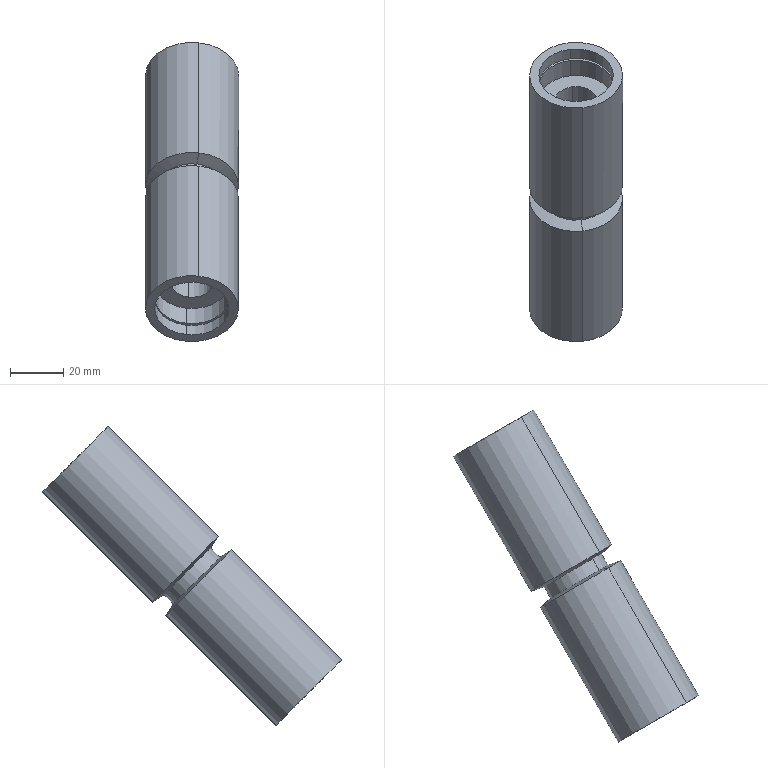Component | SolidWorks | SmallAxisAssembly-1_SmallAxisAssembly1-2_VegetablePressSmallAxisSleeve-1 | 1 solid | 32 faces | box 35.06 x 112.43 x 112.43 mm | volume 79723 mm3 | cylinder 20 | plane 8 | cone 4 | commonest cylinder face diameters 28 x8 30 x4 35 x4 16 x2 25 x2
build123d program:
from build123d import *


with BuildPart() as part:
    # Sketch1 → Revolve1 (revolve)
    with BuildSketch(Plane.XY, mode=Mode.PRIVATE) as revolve1_sk:
        Polygon((-48, 8), (48, 8), (48, 14), (56, 14), (56, 15), (57, 15), (57, 14), (62, 14), (62, 17.5), (3.5, 17.5), (2.5, 12.5), (-2.5, 12.5), (-3.5, 17.5), (-62, 17.5), (-62, 14), (-57, 14), (-57, 15), (-56, 15), (-56, 14), (-48, 14), align=None)
    revolve(revolve1_sk.sketch.rotate(Axis((-52.23, 0, 0), (1, 0, 0)), 90), axis=Axis((-52.23, 0, 0), (1, 0, 0)))


solid = part.part

# Placed as in the assembly
solid = solid.moved(Location((-41.751, 822.318, 226.866), (-134.835, -79.741, -89.832)))
STEP:
#1=CARTESIAN_POINT('',(-1.564,30.402,7.73));
#2=VERTEX_POINT('',#1);
#3=CARTESIAN_POINT('',(-1.726,31.173,6.959));
#4=VERTEX_POINT('',#3);
#5=CARTESIAN_POINT('',(-1.645,30.788,7.345));
#6=DIRECTION('',(-0.0005225,-0.7071,-0.7071));
#7=DIRECTION('',(-0.1474,0.6994,-0.6993));
#8=AXIS2_PLACEMENT_3D('',#5,#6,#7);
#9=CIRCLE('',#8,0.5512);
#10=EDGE_CURVE('',#2,#4,#9,.T.);
#11=ORIENTED_EDGE('',*,*,#10,.F.);
#12=CARTESIAN_POINT('',(-1.564,30.263,7.591));
#13=VERTEX_POINT('',#12);
#14=CARTESIAN_POINT('',(-1.564,30.535,7.863));
#15=DIRECTION('',(-0.0005225,-0.7071,-0.7071));
#16=VECTOR('',#15,39.37);
#17=LINE('',#14,#16);
#18=EDGE_CURVE('',#2,#13,#17,.T.);
#19=ORIENTED_EDGE('',*,*,#18,.T.);
#20=CARTESIAN_POINT('',(-1.726,31.034,6.82));
#21=VERTEX_POINT('',#20);
#22=CARTESIAN_POINT('',(-1.645,30.649,7.206));
#23=DIRECTION('',(-0.0005225,-0.7071,-0.7071));
#24=DIRECTION('',(-0.1474,0.6994,-0.6993));
#25=AXIS2_PLACEMENT_3D('',#22,#23,#24);
#26=CIRCLE('',#25,0.5512);
#27=EDGE_CURVE('',#13,#21,#26,.T.);
#28=ORIENTED_EDGE('',*,*,#27,.T.);
#29=CARTESIAN_POINT('',(-1.726,31.306,7.092));
#30=DIRECTION('',(-0.0005225,-0.7071,-0.7071));
#31=VECTOR('',#30,39.37);
#32=LINE('',#29,#31);
#33=EDGE_CURVE('',#4,#21,#32,.T.);
#34=ORIENTED_EDGE('',*,*,#33,.F.);
#35=EDGE_LOOP('',(#11,#19,#28,#34));
#36=FACE_OUTER_BOUND('',#35,.T.);
#37=CARTESIAN_POINT('',(-1.645,30.921,7.478));
#38=DIRECTION('',(-0.0005225,-0.7071,-0.7071));
#39=DIRECTION('',(-0.1474,0.6994,-0.6993));
#40=AXIS2_PLACEMENT_3D('',#37,#38,#39);
#41=CYLINDRICAL_SURFACE('',#40,0.5512);
#42=ADVANCED_FACE('',(#36),#41,.F.);
#43=CARTESIAN_POINT('',(-1.558,30.403,7.786));
#44=VERTEX_POINT('',#43);
#45=CARTESIAN_POINT('',(-1.732,31.229,6.96));
#46=VERTEX_POINT('',#45);
#47=CARTESIAN_POINT('',(-1.645,30.816,7.373));
#48=DIRECTION('',(-0.0005225,-0.7071,-0.7071));
#49=DIRECTION('',(-0.1474,0.6994,-0.6993));
#50=AXIS2_PLACEMENT_3D('',#47,#48,#49);
#51=CIRCLE('',#50,0.5906);
#52=EDGE_CURVE('',#44,#46,#51,.T.);
#53=ORIENTED_EDGE('',*,*,#52,.F.);
#54=CARTESIAN_POINT('',(-1.558,30.375,7.758));
#55=VERTEX_POINT('',#54);
#56=CARTESIAN_POINT('',(-1.558,30.508,7.891));
#57=DIRECTION('',(-0.0005225,-0.7071,-0.7071));
#58=VECTOR('',#57,39.37);
#59=LINE('',#56,#58);
#60=EDGE_CURVE('',#44,#55,#59,.T.);
#61=ORIENTED_EDGE('',*,*,#60,.T.);
#62=CARTESIAN_POINT('',(-1.732,31.201,6.932));
#63=VERTEX_POINT('',#62);
#64=CARTESIAN_POINT('',(-1.645,30.788,7.345));
#65=DIRECTION('',(-0.0005225,-0.7071,-0.7071));
#66=DIRECTION('',(-0.1474,0.6994,-0.6993));
#67=AXIS2_PLACEMENT_3D('',#64,#65,#66);
#68=CIRCLE('',#67,0.5906);
#69=EDGE_CURVE('',#55,#63,#68,.T.);
#70=ORIENTED_EDGE('',*,*,#69,.T.);
#71=CARTESIAN_POINT('',(-1.732,31.334,7.065));
#72=DIRECTION('',(-0.0005225,-0.7071,-0.7071));
#73=VECTOR('',#72,39.37);
#74=LINE('',#71,#73);
#75=EDGE_CURVE('',#46,#63,#74,.T.);
#76=ORIENTED_EDGE('',*,*,#75,.F.);
#77=EDGE_LOOP('',(#53,#61,#70,#76));
#78=FACE_OUTER_BOUND('',#77,.T.);
#79=CARTESIAN_POINT('',(-1.645,30.921,7.478));
#80=DIRECTION('',(-0.0005225,-0.7071,-0.7071));
#81=DIRECTION('',(-0.1474,0.6994,-0.6993));
#82=AXIS2_PLACEMENT_3D('',#79,#80,#81);
#83=CYLINDRICAL_SURFACE('',#82,0.5906);
#84=ADVANCED_FACE('',(#78),#83,.F.);
#85=CARTESIAN_POINT('',(-1.563,30.653,7.981));
#86=VERTEX_POINT('',#85);
#87=CARTESIAN_POINT('',(-1.726,31.424,7.21));
#88=VERTEX_POINT('',#87);
#89=CARTESIAN_POINT('',(-1.645,31.038,7.595));
#90=DIRECTION('',(-0.0005225,-0.7071,-0.7071));
#91=DIRECTION('',(-0.1474,0.6994,-0.6993));
#92=AXIS2_PLACEMENT_3D('',#89,#90,#91);
#93=CIRCLE('',#92,0.5512);
#94=EDGE_CURVE('',#86,#88,#93,.T.);
#95=ORIENTED_EDGE('',*,*,#94,.F.);
#96=CARTESIAN_POINT('',(-1.564,30.43,7.758));
#97=VERTEX_POINT('',#96);
#98=CARTESIAN_POINT('',(-1.564,30.535,7.863));
#99=DIRECTION('',(-0.0005225,-0.7071,-0.7071));
#100=VECTOR('',#99,39.37);
#101=LINE('',#98,#100);
#102=EDGE_CURVE('',#86,#97,#101,.T.);
#103=ORIENTED_EDGE('',*,*,#102,.T.);
#104=CARTESIAN_POINT('',(-1.726,31.201,6.987));
#105=VERTEX_POINT('',#104);
#106=CARTESIAN_POINT('',(-1.645,30.816,7.373));
#107=DIRECTION('',(-0.0005225,-0.7071,-0.7071));
#108=DIRECTION('',(-0.1474,0.6994,-0.6993));
#109=AXIS2_PLACEMENT_3D('',#106,#107,#108);
#110=CIRCLE('',#109,0.5512);
#111=EDGE_CURVE('',#97,#105,#110,.T.);
#112=ORIENTED_EDGE('',*,*,#111,.T.);
#113=CARTESIAN_POINT('',(-1.726,31.306,7.092));
#114=DIRECTION('',(-0.0005225,-0.7071,-0.7071));
#115=VECTOR('',#114,39.37);
#116=LINE('',#113,#115);
#117=EDGE_CURVE('',#88,#105,#116,.T.);
#118=ORIENTED_EDGE('',*,*,#117,.F.);
#119=EDGE_LOOP('',(#95,#103,#112,#118));
#120=FACE_OUTER_BOUND('',#119,.T.);
#121=CARTESIAN_POINT('',(-1.645,30.921,7.478));
#122=DIRECTION('',(-0.0005225,-0.7071,-0.7071));
#123=DIRECTION('',(-0.1474,0.6994,-0.6993));
#124=AXIS2_PLACEMENT_3D('',#121,#122,#123);
#125=CYLINDRICAL_SURFACE('',#124,0.5512);
#126=ADVANCED_FACE('',(#120),#125,.F.);
#127=CARTESIAN_POINT('',(-1.596,33.491,10.488));
#128=VERTEX_POINT('',#127);
#129=CARTESIAN_POINT('',(-1.689,33.931,10.048));
#130=VERTEX_POINT('',#129);
#131=CARTESIAN_POINT('',(-1.643,33.711,10.268));
#132=DIRECTION('',(-0.0005225,-0.7071,-0.7071));
#133=DIRECTION('',(-0.1474,0.6994,-0.6993));
#134=AXIS2_PLACEMENT_3D('',#131,#132,#133);
#135=CIRCLE('',#134,0.315);
#136=EDGE_CURVE('',#128,#130,#135,.T.);
#137=ORIENTED_EDGE('',*,*,#136,.F.);
#138=CARTESIAN_POINT('',(-1.598,30.818,7.816));
#139=VERTEX_POINT('',#138);
#140=CARTESIAN_POINT('',(-1.598,30.7,7.698));
#141=DIRECTION('',(-0.0005225,-0.7071,-0.7071));
#142=VECTOR('',#141,39.37);
#143=LINE('',#140,#142);
#144=EDGE_CURVE('',#128,#139,#143,.T.);
#145=ORIENTED_EDGE('',*,*,#144,.T.);
#146=CARTESIAN_POINT('',(-1.691,31.259,7.375));
#147=VERTEX_POINT('',#146);
#148=CARTESIAN_POINT('',(-1.645,31.038,7.595));
#149=DIRECTION('',(-0.0005225,-0.7071,-0.7071));
#150=DIRECTION('',(-0.1474,0.6994,-0.6993));
#151=AXIS2_PLACEMENT_3D('',#148,#149,#150);
#152=CIRCLE('',#151,0.315);
#153=EDGE_CURVE('',#139,#147,#152,.T.);
#154=ORIENTED_EDGE('',*,*,#153,.T.);
#155=CARTESIAN_POINT('',(-1.691,31.141,7.257));
#156=DIRECTION('',(-0.0005225,-0.7071,-0.7071));
#157=VECTOR('',#156,39.37);
#158=LINE('',#155,#157);
#159=EDGE_CURVE('',#130,#147,#158,.T.);
#160=ORIENTED_EDGE('',*,*,#159,.F.);
#161=EDGE_LOOP('',(#137,#145,#154,#160));
#162=FACE_OUTER_BOUND('',#161,.T.);
#163=CARTESIAN_POINT('',(-1.645,30.921,7.478));
#164=DIRECTION('',(-0.0005225,-0.7071,-0.7071));
#165=DIRECTION('',(-0.1474,0.6994,-0.6993));
#166=AXIS2_PLACEMENT_3D('',#163,#164,#165);
#167=CYLINDRICAL_SURFACE('',#166,0.315);
#168=ADVANCED_FACE('',(#162),#167,.F.);
#169=CARTESIAN_POINT('',(-1.561,33.548,10.876));
#170=VERTEX_POINT('',#169);
#171=CARTESIAN_POINT('',(-1.724,34.319,10.105));
#172=VERTEX_POINT('',#171);
#173=CARTESIAN_POINT('',(-1.643,33.934,10.491));
#174=DIRECTION('',(-0.0005225,-0.7071,-0.7071));
#175=DIRECTION('',(-0.1474,0.6994,-0.6993));
#176=AXIS2_PLACEMENT_3D('',#173,#174,#175);
#177=CIRCLE('',#176,0.5512);
#178=EDGE_CURVE('',#170,#172,#177,.T.);
#179=ORIENTED_EDGE('',*,*,#178,.F.);
#180=CARTESIAN_POINT('',(-1.562,33.325,10.653));
#181=VERTEX_POINT('',#180);
#182=CARTESIAN_POINT('',(-1.564,30.535,7.863));
#183=DIRECTION('',(-0.0005225,-0.7071,-0.7071));
#184=VECTOR('',#183,39.37);
#185=LINE('',#182,#184);
#186=EDGE_CURVE('',#170,#181,#185,.T.);
#187=ORIENTED_EDGE('',*,*,#186,.T.);
#188=CARTESIAN_POINT('',(-1.724,34.097,9.883));
#189=VERTEX_POINT('',#188);
#190=CARTESIAN_POINT('',(-1.643,33.711,10.268));
#191=DIRECTION('',(-0.0005225,-0.7071,-0.7071));
#192=DIRECTION('',(-0.1474,0.6994,-0.6993));
#193=AXIS2_PLACEMENT_3D('',#190,#191,#192);
#194=CIRCLE('',#193,0.5512);
#195=EDGE_CURVE('',#181,#189,#194,.T.);
#196=ORIENTED_EDGE('',*,*,#195,.T.);
#197=CARTESIAN_POINT('',(-1.726,31.306,7.092));
#198=DIRECTION('',(-0.0005225,-0.7071,-0.7071));
#199=VECTOR('',#198,39.37);
#200=LINE('',#197,#199);
#201=EDGE_CURVE('',#172,#189,#200,.T.);
#202=ORIENTED_EDGE('',*,*,#201,.F.);
#203=EDGE_LOOP('',(#179,#187,#196,#202));
#204=FACE_OUTER_BOUND('',#203,.T.);
#205=CARTESIAN_POINT('',(-1.645,30.921,7.478));
#206=DIRECTION('',(-0.0005225,-0.7071,-0.7071));
#207=DIRECTION('',(-0.1474,0.6994,-0.6993));
#208=AXIS2_PLACEMENT_3D('',#205,#206,#207);
#209=CYLINDRICAL_SURFACE('',#208,0.5512);
#210=ADVANCED_FACE('',(#204),#209,.F.);
#211=CARTESIAN_POINT('',(-1.556,33.548,10.932));
#212=VERTEX_POINT('',#211);
#213=CARTESIAN_POINT('',(-1.73,34.375,10.106));
#214=VERTEX_POINT('',#213);
#215=CARTESIAN_POINT('',(-1.643,33.962,10.519));
#216=DIRECTION('',(-0.0005225,-0.7071,-0.7071));
#217=DIRECTION('',(-0.1474,0.6994,-0.6993));
#218=AXIS2_PLACEMENT_3D('',#215,#216,#217);
#219=CIRCLE('',#218,0.5906);
#220=EDGE_CURVE('',#212,#214,#219,.T.);
#221=ORIENTED_EDGE('',*,*,#220,.F.);
#222=CARTESIAN_POINT('',(-1.556,33.521,10.904));
#223=VERTEX_POINT('',#222);
#224=CARTESIAN_POINT('',(-1.558,30.508,7.891));
#225=DIRECTION('',(-0.0005225,-0.7071,-0.7071));
#226=VECTOR('',#225,39.37);
#227=LINE('',#224,#226);
#228=EDGE_CURVE('',#212,#223,#227,.T.);
#229=ORIENTED_EDGE('',*,*,#228,.T.);
#230=CARTESIAN_POINT('',(-1.73,34.347,10.078));
#231=VERTEX_POINT('',#230);
#232=CARTESIAN_POINT('',(-1.643,33.934,10.491));
#233=DIRECTION('',(-0.0005225,-0.7071,-0.7071));
#234=DIRECTION('',(-0.1474,0.6994,-0.6993));
#235=AXIS2_PLACEMENT_3D('',#232,#233,#234);
#236=CIRCLE('',#235,0.5906);
#237=EDGE_CURVE('',#223,#231,#236,.T.);
#238=ORIENTED_EDGE('',*,*,#237,.T.);
#239=CARTESIAN_POINT('',(-1.732,31.334,7.065));
#240=DIRECTION('',(-0.0005225,-0.7071,-0.7071));
#241=VECTOR('',#240,39.37);
#242=LINE('',#239,#241);
#243=EDGE_CURVE('',#214,#231,#242,.T.);
#244=ORIENTED_EDGE('',*,*,#243,.F.);
#245=EDGE_LOOP('',(#221,#229,#238,#244));
#246=FACE_OUTER_BOUND('',#245,.T.);
#247=CARTESIAN_POINT('',(-1.645,30.921,7.478));
#248=DIRECTION('',(-0.0005225,-0.7071,-0.7071));
#249=DIRECTION('',(-0.1474,0.6994,-0.6993));
#250=AXIS2_PLACEMENT_3D('',#247,#248,#249);
#251=CYLINDRICAL_SURFACE('',#250,0.5906);
#252=ADVANCED_FACE('',(#246),#251,.F.);
#253=CARTESIAN_POINT('',(-1.561,33.715,11.043));
#254=VERTEX_POINT('',#253);
#255=CARTESIAN_POINT('',(-1.724,34.486,10.272));
#256=VERTEX_POINT('',#255);
#257=CARTESIAN_POINT('',(-1.642,34.101,10.658));
#258=DIRECTION('',(-0.0005225,-0.7071,-0.7071));
#259=DIRECTION('',(-0.1474,0.6994,-0.6993));
#260=AXIS2_PLACEMENT_3D('',#257,#258,#259);
#261=CIRCLE('',#260,0.5512);
#262=EDGE_CURVE('',#254,#256,#261,.T.);
#263=ORIENTED_EDGE('',*,*,#262,.F.);
#264=CARTESIAN_POINT('',(-1.561,33.576,10.904));
#265=VERTEX_POINT('',#264);
#266=CARTESIAN_POINT('',(-1.564,30.535,7.863));
#267=DIRECTION('',(-0.0005225,-0.7071,-0.7071));
#268=VECTOR('',#267,39.37);
#269=LINE('',#266,#268);
#270=EDGE_CURVE('',#254,#265,#269,.T.);
#271=ORIENTED_EDGE('',*,*,#270,.T.);
#272=CARTESIAN_POINT('',(-1.724,34.347,10.133));
#273=VERTEX_POINT('',#272);
#274=CARTESIAN_POINT('',(-1.643,33.962,10.519));
#275=DIRECTION('',(-0.0005225,-0.7071,-0.7071));
#276=DIRECTION('',(-0.1474,0.6994,-0.6993));
#277=AXIS2_PLACEMENT_3D('',#274,#275,#276);
#278=CIRCLE('',#277,0.5512);
#279=EDGE_CURVE('',#265,#273,#278,.T.);
#280=ORIENTED_EDGE('',*,*,#279,.T.);
#281=CARTESIAN_POINT('',(-1.726,31.306,7.092));
#282=DIRECTION('',(-0.0005225,-0.7071,-0.7071));
#283=VECTOR('',#282,39.37);
#284=LINE('',#281,#283);
#285=EDGE_CURVE('',#256,#273,#284,.T.);
#286=ORIENTED_EDGE('',*,*,#285,.F.);
#287=EDGE_LOOP('',(#263,#271,#280,#286));
#288=FACE_OUTER_BOUND('',#287,.T.);
#289=CARTESIAN_POINT('',(-1.645,30.921,7.478));
#290=DIRECTION('',(-0.0005225,-0.7071,-0.7071));
#291=DIRECTION('',(-0.1474,0.6994,-0.6993));
#292=AXIS2_PLACEMENT_3D('',#289,#290,#291);
#293=CYLINDRICAL_SURFACE('',#292,0.5512);
#294=ADVANCED_FACE('',(#288),#293,.F.);
#295=CARTESIAN_POINT('',(-1.744,34.583,10.176));
#296=VERTEX_POINT('',#295);
#297=CARTESIAN_POINT('',(-1.541,33.619,11.14));
#298=VERTEX_POINT('',#297);
#299=CARTESIAN_POINT('',(-1.642,34.101,10.658));
#300=DIRECTION('',(-0.0005225,-0.7071,-0.7071));
#301=DIRECTION('',(-0.1474,0.6994,-0.6993));
#302=AXIS2_PLACEMENT_3D('',#299,#300,#301);
#303=CIRCLE('',#302,0.689);
#304=EDGE_CURVE('',#296,#298,#303,.T.);
#305=ORIENTED_EDGE('',*,*,#304,.T.);
#306=CARTESIAN_POINT('',(-1.542,31.99,9.511));
#307=VERTEX_POINT('',#306);
#308=CARTESIAN_POINT('',(-1.543,30.439,7.96));
#309=DIRECTION('',(-0.0005225,-0.7071,-0.7071));
#310=VECTOR('',#309,39.37);
#311=LINE('',#308,#310);
#312=EDGE_CURVE('',#298,#307,#311,.T.);
#313=ORIENTED_EDGE('',*,*,#312,.T.);
#314=CARTESIAN_POINT('',(-1.745,32.954,8.547));
#315=VERTEX_POINT('',#314);
#316=CARTESIAN_POINT('',(-1.644,32.472,9.029));
#317=DIRECTION('',(-0.0005225,-0.7071,-0.7071));
#318=DIRECTION('',(-0.1474,0.6994,-0.6993));
#319=AXIS2_PLACEMENT_3D('',#316,#317,#318);
#320=CIRCLE('',#319,0.689);
#321=EDGE_CURVE('',#315,#307,#320,.T.);
#322=ORIENTED_EDGE('',*,*,#321,.F.);
#323=CARTESIAN_POINT('',(-1.746,31.403,6.996));
#324=DIRECTION('',(-0.0005225,-0.7071,-0.7071));
#325=VECTOR('',#324,39.37);
#326=LINE('',#323,#325);
#327=EDGE_CURVE('',#296,#315,#326,.T.);
#328=ORIENTED_EDGE('',*,*,#327,.F.);
#329=EDGE_LOOP('',(#305,#313,#322,#328));
#330=FACE_OUTER_BOUND('',#329,.T.);
#331=CARTESIAN_POINT('',(-1.645,30.921,7.478));
#332=DIRECTION('',(-0.0005225,-0.7071,-0.7071));
#333=DIRECTION('',(-0.1474,0.6994,-0.6993));
#334=AXIS2_PLACEMENT_3D('',#331,#332,#333);
#335=CYLINDRICAL_SURFACE('',#334,0.689);
#336=ADVANCED_FACE('',(#330),#335,.T.);
#337=CARTESIAN_POINT('',(-1.716,32.789,8.657));
#338=VERTEX_POINT('',#337);
#339=CARTESIAN_POINT('',(-1.571,32.1,9.345));
#340=VERTEX_POINT('',#339);
#341=CARTESIAN_POINT('',(-1.644,32.444,9.001));
#342=DIRECTION('',(-0.0005225,-0.7071,-0.7071));
#343=DIRECTION('',(-0.1474,0.6994,-0.6993));
#344=AXIS2_PLACEMENT_3D('',#341,#342,#343);
#345=CIRCLE('',#344,0.4921);
#346=EDGE_CURVE('',#338,#340,#345,.T.);
#347=ORIENTED_EDGE('',*,*,#346,.F.);
#348=CARTESIAN_POINT('',(-1.745,32.954,8.547));
#349=DIRECTION('',(-0.1444,0.8245,-0.5471));
#350=VECTOR('',#349,39.37);
#351=LINE('',#348,#350);
#352=EDGE_CURVE('',#338,#315,#351,.T.);
#353=ORIENTED_EDGE('',*,*,#352,.T.);
#354=ORIENTED_EDGE('',*,*,#321,.T.);
#355=CARTESIAN_POINT('',(-1.542,31.99,9.511));
#356=DIRECTION('',(0.1447,-0.5472,0.8244));
#357=VECTOR('',#356,39.37);
#358=LINE('',#355,#357);
#359=EDGE_CURVE('',#340,#307,#358,.T.);
#360=ORIENTED_EDGE('',*,*,#359,.F.);
#361=EDGE_LOOP('',(#347,#353,#354,#360));
#362=FACE_OUTER_BOUND('',#361,.T.);
#363=CARTESIAN_POINT('',(-1.644,32.472,9.029));
#364=DIRECTION('',(0.0005225,0.7071,0.7071));
#365=DIRECTION('',(0.1474,-0.6994,0.6993));
#366=AXIS2_PLACEMENT_3D('',#363,#364,#365);
#367=CONICAL_SURFACE('',#366,0.689,1.373);
#368=ADVANCED_FACE('',(#362),#367,.T.);
#369=ORIENTED_EDGE('',*,*,#346,.T.);
#370=CARTESIAN_POINT('',(-1.571,31.961,9.206));
#371=VERTEX_POINT('',#370);
#372=CARTESIAN_POINT('',(-1.572,30.576,7.822));
#373=DIRECTION('',(-0.0005225,-0.7071,-0.7071));
#374=VECTOR('',#373,39.37);
#375=LINE('',#372,#374);
#376=EDGE_CURVE('',#340,#371,#375,.T.);
#377=ORIENTED_EDGE('',*,*,#376,.T.);
#378=CARTESIAN_POINT('',(-1.716,32.649,8.518));
#379=VERTEX_POINT('',#378);
#380=CARTESIAN_POINT('',(-1.644,32.305,8.862));
#381=DIRECTION('',(-0.0005225,-0.7071,-0.7071));
#382=DIRECTION('',(-0.1474,0.6994,-0.6993));
#383=AXIS2_PLACEMENT_3D('',#380,#381,#382);
#384=CIRCLE('',#383,0.4921);
#385=EDGE_CURVE('',#379,#371,#384,.T.);
#386=ORIENTED_EDGE('',*,*,#385,.F.);
#387=CARTESIAN_POINT('',(-1.717,31.265,7.134));
#388=DIRECTION('',(-0.0005225,-0.7071,-0.7071));
#389=VECTOR('',#388,39.37);
#390=LINE('',#387,#389);
#391=EDGE_CURVE('',#338,#379,#390,.T.);
#392=ORIENTED_EDGE('',*,*,#391,.F.);
#393=EDGE_LOOP('',(#369,#377,#386,#392));
#394=FACE_OUTER_BOUND('',#393,.T.);
#395=CARTESIAN_POINT('',(-1.645,30.921,7.478));
#396=DIRECTION('',(-0.0005225,-0.7071,-0.7071));
#397=DIRECTION('',(-0.1474,0.6994,-0.6993));
#398=AXIS2_PLACEMENT_3D('',#395,#396,#397);
#399=CYLINDRICAL_SURFACE('',#398,0.4921);
#400=ADVANCED_FACE('',(#394),#399,.T.);
#401=ORIENTED_EDGE('',*,*,#385,.T.);
#402=CARTESIAN_POINT('',(-1.542,31.795,9.316));
#403=VERTEX_POINT('',#402);
#404=CARTESIAN_POINT('',(-1.571,31.961,9.206));
#405=DIRECTION('',(0.1444,-0.8245,0.5471));
#406=VECTOR('',#405,39.37);
#407=LINE('',#404,#406);
#408=EDGE_CURVE('',#371,#403,#407,.T.);
#409=ORIENTED_EDGE('',*,*,#408,.T.);
#410=CARTESIAN_POINT('',(-1.745,32.759,8.352));
#411=VERTEX_POINT('',#410);
#412=CARTESIAN_POINT('',(-1.644,32.277,8.834));
#413=DIRECTION('',(-0.0005225,-0.7071,-0.7071));
#414=DIRECTION('',(-0.1474,0.6994,-0.6993));
#415=AXIS2_PLACEMENT_3D('',#412,#413,#414);
#416=CIRCLE('',#415,0.689);
#417=EDGE_CURVE('',#411,#403,#416,.T.);
#418=ORIENTED_EDGE('',*,*,#417,.F.);
#419=CARTESIAN_POINT('',(-1.716,32.649,8.518));
#420=DIRECTION('',(-0.1447,0.5472,-0.8244));
#421=VECTOR('',#420,39.37);
#422=LINE('',#419,#421);
#423=EDGE_CURVE('',#379,#411,#422,.T.);
#424=ORIENTED_EDGE('',*,*,#423,.F.);
#425=EDGE_LOOP('',(#401,#409,#418,#424));
#426=FACE_OUTER_BOUND('',#425,.T.);
#427=CARTESIAN_POINT('',(-1.644,32.305,8.862));
#428=DIRECTION('',(-0.0005225,-0.7071,-0.7071));
#429=DIRECTION('',(-0.1474,0.6994,-0.6993));
#430=AXIS2_PLACEMENT_3D('',#427,#428,#429);
#431=CONICAL_SURFACE('',#430,0.4921,1.373);
#432=ADVANCED_FACE('',(#426),#431,.T.);
#433=ORIENTED_EDGE('',*,*,#417,.T.);
#434=CARTESIAN_POINT('',(-1.543,30.167,7.688));
#435=VERTEX_POINT('',#434);
#436=CARTESIAN_POINT('',(-1.543,30.439,7.96));
#437=DIRECTION('',(-0.0005225,-0.7071,-0.7071));
#438=VECTOR('',#437,39.37);
#439=LINE('',#436,#438);
#440=EDGE_CURVE('',#403,#435,#439,.T.);
#441=ORIENTED_EDGE('',*,*,#440,.T.);
#442=CARTESIAN_POINT('',(-1.747,31.131,6.724));
#443=VERTEX_POINT('',#442);
#444=CARTESIAN_POINT('',(-1.645,30.649,7.206));
#445=DIRECTION('',(-0.0005225,-0.7071,-0.7071));
#446=DIRECTION('',(-0.1474,0.6994,-0.6993));
#447=AXIS2_PLACEMENT_3D('',#444,#445,#446);
#448=CIRCLE('',#447,0.689);
#449=EDGE_CURVE('',#443,#435,#448,.T.);
#450=ORIENTED_EDGE('',*,*,#449,.F.);
#451=CARTESIAN_POINT('',(-1.746,31.403,6.996));
#452=DIRECTION('',(-0.0005225,-0.7071,-0.7071));
#453=VECTOR('',#452,39.37);
#454=LINE('',#451,#453);
#455=EDGE_CURVE('',#411,#443,#454,.T.);
#456=ORIENTED_EDGE('',*,*,#455,.F.);
#457=EDGE_LOOP('',(#433,#441,#450,#456));
#458=FACE_OUTER_BOUND('',#457,.T.);
#459=CARTESIAN_POINT('',(-1.645,30.921,7.478));
#460=DIRECTION('',(-0.0005225,-0.7071,-0.7071));
#461=DIRECTION('',(-0.1474,0.6994,-0.6993));
#462=AXIS2_PLACEMENT_3D('',#459,#460,#461);
#463=CYLINDRICAL_SURFACE('',#462,0.689);
#464=ADVANCED_FACE('',(#458),#463,.T.);
#465=ORIENTED_EDGE('',*,*,#440,.F.);
#466=CARTESIAN_POINT('',(-1.644,32.277,8.834));
#467=DIRECTION('',(-0.0005225,-0.7071,-0.7071));
#468=DIRECTION('',(-0.1474,0.6994,-0.6993));
#469=AXIS2_PLACEMENT_3D('',#466,#467,#468);
#470=CIRCLE('',#469,0.689);
#471=EDGE_CURVE('',#403,#411,#470,.T.);
#472=ORIENTED_EDGE('',*,*,#471,.T.);
#473=ORIENTED_EDGE('',*,*,#455,.T.);
#474=CARTESIAN_POINT('',(-1.645,30.649,7.206));
#475=DIRECTION('',(-0.0005225,-0.7071,-0.7071));
#476=DIRECTION('',(-0.1474,0.6994,-0.6993));
#477=AXIS2_PLACEMENT_3D('',#474,#475,#476);
#478=CIRCLE('',#477,0.689);
#479=EDGE_CURVE('',#435,#443,#478,.T.);
#480=ORIENTED_EDGE('',*,*,#479,.F.);
#481=EDGE_LOOP('',(#465,#472,#473,#480));
#482=FACE_OUTER_BOUND('',#481,.T.);
#483=CARTESIAN_POINT('',(-1.645,30.921,7.478));
#484=DIRECTION('',(-0.0005225,-0.7071,-0.7071));
#485=DIRECTION('',(-0.1474,0.6994,-0.6993));
#486=AXIS2_PLACEMENT_3D('',#483,#484,#485);
#487=CYLINDRICAL_SURFACE('',#486,0.689);
#488=ADVANCED_FACE('',(#482),#487,.T.);
#489=ORIENTED_EDGE('',*,*,#408,.F.);
#490=CARTESIAN_POINT('',(-1.644,32.305,8.862));
#491=DIRECTION('',(-0.0005225,-0.7071,-0.7071));
#492=DIRECTION('',(-0.1474,0.6994,-0.6993));
#493=AXIS2_PLACEMENT_3D('',#490,#491,#492);
#494=CIRCLE('',#493,0.4921);
#495=EDGE_CURVE('',#371,#379,#494,.T.);
#496=ORIENTED_EDGE('',*,*,#495,.T.);
#497=ORIENTED_EDGE('',*,*,#423,.T.);
#498=ORIENTED_EDGE('',*,*,#471,.F.);
#499=EDGE_LOOP('',(#489,#496,#497,#498));
#500=FACE_OUTER_BOUND('',#499,.T.);
#501=CARTESIAN_POINT('',(-1.644,32.305,8.862));
#502=DIRECTION('',(-0.0005225,-0.7071,-0.7071));
#503=DIRECTION('',(-0.1474,0.6994,-0.6993));
#504=AXIS2_PLACEMENT_3D('',#501,#502,#503);
#505=CONICAL_SURFACE('',#504,0.4921,1.373);
#506=ADVANCED_FACE('',(#500),#505,.T.);
#507=ORIENTED_EDGE('',*,*,#376,.F.);
#508=CARTESIAN_POINT('',(-1.644,32.444,9.001));
#509=DIRECTION('',(-0.0005225,-0.7071,-0.7071));
#510=DIRECTION('',(-0.1474,0.6994,-0.6993));
#511=AXIS2_PLACEMENT_3D('',#508,#509,#510);
#512=CIRCLE('',#511,0.4921);
#513=EDGE_CURVE('',#340,#338,#512,.T.);
#514=ORIENTED_EDGE('',*,*,#513,.T.);
#515=ORIENTED_EDGE('',*,*,#391,.T.);
#516=ORIENTED_EDGE('',*,*,#495,.F.);
#517=EDGE_LOOP('',(#507,#514,#515,#516));
#518=FACE_OUTER_BOUND('',#517,.T.);
#519=CARTESIAN_POINT('',(-1.645,30.921,7.478));
#520=DIRECTION('',(-0.0005225,-0.7071,-0.7071));
#521=DIRECTION('',(-0.1474,0.6994,-0.6993));
#522=AXIS2_PLACEMENT_3D('',#519,#520,#521);
#523=CYLINDRICAL_SURFACE('',#522,0.4921);
#524=ADVANCED_FACE('',(#518),#523,.T.);
#525=ORIENTED_EDGE('',*,*,#352,.F.);
#526=ORIENTED_EDGE('',*,*,#513,.F.);
#527=ORIENTED_EDGE('',*,*,#359,.T.);
#528=CARTESIAN_POINT('',(-1.644,32.472,9.029));
#529=DIRECTION('',(-0.0005225,-0.7071,-0.7071));
#530=DIRECTION('',(-0.1474,0.6994,-0.6993));
#531=AXIS2_PLACEMENT_3D('',#528,#529,#530);
#532=CIRCLE('',#531,0.689);
#533=EDGE_CURVE('',#307,#315,#532,.T.);
#534=ORIENTED_EDGE('',*,*,#533,.T.);
#535=EDGE_LOOP('',(#525,#526,#527,#534));
#536=FACE_OUTER_BOUND('',#535,.T.);
#537=CARTESIAN_POINT('',(-1.644,32.472,9.029));
#538=DIRECTION('',(0.0005225,0.7071,0.7071));
#539=DIRECTION('',(0.1474,-0.6994,0.6993));
#540=AXIS2_PLACEMENT_3D('',#537,#538,#539);
#541=CONICAL_SURFACE('',#540,0.689,1.373);
#542=ADVANCED_FACE('',(#536),#541,.T.);
#543=ORIENTED_EDGE('',*,*,#312,.F.);
#544=CARTESIAN_POINT('',(-1.642,34.101,10.658));
#545=DIRECTION('',(-0.0005225,-0.7071,-0.7071));
#546=DIRECTION('',(-0.1474,0.6994,-0.6993));
#547=AXIS2_PLACEMENT_3D('',#544,#545,#546);
#548=CIRCLE('',#547,0.689);
#549=EDGE_CURVE('',#298,#296,#548,.T.);
#550=ORIENTED_EDGE('',*,*,#549,.T.);
#551=ORIENTED_EDGE('',*,*,#327,.T.);
#552=ORIENTED_EDGE('',*,*,#533,.F.);
#553=EDGE_LOOP('',(#543,#550,#551,#552));
#554=FACE_OUTER_BOUND('',#553,.T.);
#555=CARTESIAN_POINT('',(-1.645,30.921,7.478));
#556=DIRECTION('',(-0.0005225,-0.7071,-0.7071));
#557=DIRECTION('',(-0.1474,0.6994,-0.6993));
#558=AXIS2_PLACEMENT_3D('',#555,#556,#557);
#559=CYLINDRICAL_SURFACE('',#558,0.689);
#560=ADVANCED_FACE('',(#554),#559,.T.);
#561=ORIENTED_EDGE('',*,*,#304,.F.);
#562=ORIENTED_EDGE('',*,*,#549,.F.);
#563=EDGE_LOOP('',(#561,#562));
#564=FACE_OUTER_BOUND('',#563,.T.);
#565=CARTESIAN_POINT('',(-1.642,34.101,10.658));
#566=DIRECTION('',(-0.0005225,-0.7071,-0.7071));
#567=DIRECTION('',(-0.1474,0.6994,-0.6993));
#568=AXIS2_PLACEMENT_3D('',#565,#566,#567);
#569=CIRCLE('',#568,0.5512);
#570=EDGE_CURVE('',#256,#254,#569,.T.);
#571=ORIENTED_EDGE('',*,*,#570,.T.);
#572=ORIENTED_EDGE('',*,*,#262,.T.);
#573=EDGE_LOOP('',(#571,#572));
#574=FACE_BOUND('',#573,.T.);
#575=CARTESIAN_POINT('',(-1.097,34.158,10.6));
#576=DIRECTION('',(-0.0005225,-0.7071,-0.7071));
#577=DIRECTION('',(-0.1474,0.6994,-0.6993));
#578=AXIS2_PLACEMENT_3D('',#575,#576,#577);
#579=PLANE('',#578);
#580=ADVANCED_FACE('',(#564,#574),#579,.F.);
#581=ORIENTED_EDGE('',*,*,#270,.F.);
#582=ORIENTED_EDGE('',*,*,#570,.F.);
#583=ORIENTED_EDGE('',*,*,#285,.T.);
#584=CARTESIAN_POINT('',(-1.643,33.962,10.519));
#585=DIRECTION('',(-0.0005225,-0.7071,-0.7071));
#586=DIRECTION('',(-0.1474,0.6994,-0.6993));
#587=AXIS2_PLACEMENT_3D('',#584,#585,#586);
#588=CIRCLE('',#587,0.5512);
#589=EDGE_CURVE('',#273,#265,#588,.T.);
#590=ORIENTED_EDGE('',*,*,#589,.T.);
#591=EDGE_LOOP('',(#581,#582,#583,#590));
#592=FACE_OUTER_BOUND('',#591,.T.);
#593=CARTESIAN_POINT('',(-1.645,30.921,7.478));
#594=DIRECTION('',(-0.0005225,-0.7071,-0.7071));
#595=DIRECTION('',(-0.1474,0.6994,-0.6993));
#596=AXIS2_PLACEMENT_3D('',#593,#594,#595);
#597=CYLINDRICAL_SURFACE('',#596,0.5512);
#598=ADVANCED_FACE('',(#592),#597,.F.);
#599=ORIENTED_EDGE('',*,*,#589,.F.);
#600=ORIENTED_EDGE('',*,*,#279,.F.);
#601=EDGE_LOOP('',(#599,#600));
#602=FACE_BOUND('',#601,.T.);
#603=CARTESIAN_POINT('',(-1.643,33.962,10.519));
#604=DIRECTION('',(-0.0005225,-0.7071,-0.7071));
#605=DIRECTION('',(-0.1474,0.6994,-0.6993));
#606=AXIS2_PLACEMENT_3D('',#603,#604,#605);
#607=CIRCLE('',#606,0.5906);
#608=EDGE_CURVE('',#214,#212,#607,.T.);
#609=ORIENTED_EDGE('',*,*,#608,.T.);
#610=ORIENTED_EDGE('',*,*,#220,.T.);
#611=EDGE_LOOP('',(#609,#610));
#612=FACE_OUTER_BOUND('',#611,.T.);
#613=CARTESIAN_POINT('',(-1.058,34.023,10.457));
#614=DIRECTION('',(0.0005225,0.7071,0.7071));
#615=DIRECTION('',(0.1474,-0.6994,0.6993));
#616=AXIS2_PLACEMENT_3D('',#613,#614,#615);
#617=PLANE('',#616);
#618=ADVANCED_FACE('',(#602,#612),#617,.F.);
#619=ORIENTED_EDGE('',*,*,#228,.F.);
#620=ORIENTED_EDGE('',*,*,#608,.F.);
#621=ORIENTED_EDGE('',*,*,#243,.T.);
#622=CARTESIAN_POINT('',(-1.643,33.934,10.491));
#623=DIRECTION('',(-0.0005225,-0.7071,-0.7071));
#624=DIRECTION('',(-0.1474,0.6994,-0.6993));
#625=AXIS2_PLACEMENT_3D('',#622,#623,#624);
#626=CIRCLE('',#625,0.5906);
#627=EDGE_CURVE('',#231,#223,#626,.T.);
#628=ORIENTED_EDGE('',*,*,#627,.T.);
#629=EDGE_LOOP('',(#619,#620,#621,#628));
#630=FACE_OUTER_BOUND('',#629,.T.);
#631=CARTESIAN_POINT('',(-1.645,30.921,7.478));
#632=DIRECTION('',(-0.0005225,-0.7071,-0.7071));
#633=DIRECTION('',(-0.1474,0.6994,-0.6993));
#634=AXIS2_PLACEMENT_3D('',#631,#632,#633);
#635=CYLINDRICAL_SURFACE('',#634,0.5906);
#636=ADVANCED_FACE('',(#630),#635,.F.);
#637=ORIENTED_EDGE('',*,*,#627,.F.);
#638=ORIENTED_EDGE('',*,*,#237,.F.);
#639=EDGE_LOOP('',(#637,#638));
#640=FACE_OUTER_BOUND('',#639,.T.);
#641=CARTESIAN_POINT('',(-1.643,33.934,10.491));
#642=DIRECTION('',(-0.0005225,-0.7071,-0.7071));
#643=DIRECTION('',(-0.1474,0.6994,-0.6993));
#644=AXIS2_PLACEMENT_3D('',#641,#642,#643);
#645=CIRCLE('',#644,0.5512);
#646=EDGE_CURVE('',#172,#170,#645,.T.);
#647=ORIENTED_EDGE('',*,*,#646,.T.);
#648=ORIENTED_EDGE('',*,*,#178,.T.);
#649=EDGE_LOOP('',(#647,#648));
#650=FACE_BOUND('',#649,.T.);
#651=CARTESIAN_POINT('',(-1.097,33.991,10.433));
#652=DIRECTION('',(-0.0005225,-0.7071,-0.7071));
#653=DIRECTION('',(-0.1474,0.6994,-0.6993));
#654=AXIS2_PLACEMENT_3D('',#651,#652,#653);
#655=PLANE('',#654);
#656=ADVANCED_FACE('',(#640,#650),#655,.F.);
#657=ORIENTED_EDGE('',*,*,#186,.F.);
#658=ORIENTED_EDGE('',*,*,#646,.F.);
#659=ORIENTED_EDGE('',*,*,#201,.T.);
#660=CARTESIAN_POINT('',(-1.643,33.711,10.268));
#661=DIRECTION('',(-0.0005225,-0.7071,-0.7071));
#662=DIRECTION('',(-0.1474,0.6994,-0.6993));
#663=AXIS2_PLACEMENT_3D('',#660,#661,#662);
#664=CIRCLE('',#663,0.5512);
#665=EDGE_CURVE('',#189,#181,#664,.T.);
#666=ORIENTED_EDGE('',*,*,#665,.T.);
#667=EDGE_LOOP('',(#657,#658,#659,#666));
#668=FACE_OUTER_BOUND('',#667,.T.);
#669=CARTESIAN_POINT('',(-1.645,30.921,7.478));
#670=DIRECTION('',(-0.0005225,-0.7071,-0.7071));
#671=DIRECTION('',(-0.1474,0.6994,-0.6993));
#672=AXIS2_PLACEMENT_3D('',#669,#670,#671);
#673=CYLINDRICAL_SURFACE('',#672,0.5512);
#674=ADVANCED_FACE('',(#668),#673,.F.);
#675=ORIENTED_EDGE('',*,*,#665,.F.);
#676=ORIENTED_EDGE('',*,*,#195,.F.);
#677=EDGE_LOOP('',(#675,#676));
#678=FACE_OUTER_BOUND('',#677,.T.);
#679=CARTESIAN_POINT('',(-1.643,33.711,10.268));
#680=DIRECTION('',(-0.0005225,-0.7071,-0.7071));
#681=DIRECTION('',(-0.1474,0.6994,-0.6993));
#682=AXIS2_PLACEMENT_3D('',#679,#680,#681);
#683=CIRCLE('',#682,0.315);
#684=EDGE_CURVE('',#130,#128,#683,.T.);
#685=ORIENTED_EDGE('',*,*,#684,.T.);
#686=ORIENTED_EDGE('',*,*,#136,.T.);
#687=EDGE_LOOP('',(#685,#686));
#688=FACE_BOUND('',#687,.T.);
#689=CARTESIAN_POINT('',(-1.331,33.744,10.235));
#690=DIRECTION('',(-0.0005225,-0.7071,-0.7071));
#691=DIRECTION('',(-0.1474,0.6994,-0.6993));
#692=AXIS2_PLACEMENT_3D('',#689,#690,#691);
#693=PLANE('',#692);
#694=ADVANCED_FACE('',(#678,#688),#693,.F.);
#695=ORIENTED_EDGE('',*,*,#144,.F.);
#696=ORIENTED_EDGE('',*,*,#684,.F.);
#697=ORIENTED_EDGE('',*,*,#159,.T.);
#698=CARTESIAN_POINT('',(-1.645,31.038,7.595));
#699=DIRECTION('',(-0.0005225,-0.7071,-0.7071));
#700=DIRECTION('',(-0.1474,0.6994,-0.6993));
#701=AXIS2_PLACEMENT_3D('',#698,#699,#700);
#702=CIRCLE('',#701,0.315);
#703=EDGE_CURVE('',#147,#139,#702,.T.);
#704=ORIENTED_EDGE('',*,*,#703,.T.);
#705=EDGE_LOOP('',(#695,#696,#697,#704));
#706=FACE_OUTER_BOUND('',#705,.T.);
#707=CARTESIAN_POINT('',(-1.645,30.921,7.478));
#708=DIRECTION('',(-0.0005225,-0.7071,-0.7071));
#709=DIRECTION('',(-0.1474,0.6994,-0.6993));
#710=AXIS2_PLACEMENT_3D('',#707,#708,#709);
#711=CYLINDRICAL_SURFACE('',#710,0.315);
#712=ADVANCED_FACE('',(#706),#711,.F.);
#713=ORIENTED_EDGE('',*,*,#703,.F.);
#714=ORIENTED_EDGE('',*,*,#153,.F.);
#715=EDGE_LOOP('',(#713,#714));
#716=FACE_BOUND('',#715,.T.);
#717=CARTESIAN_POINT('',(-1.645,31.038,7.595));
#718=DIRECTION('',(-0.0005225,-0.7071,-0.7071));
#719=DIRECTION('',(-0.1474,0.6994,-0.6993));
#720=AXIS2_PLACEMENT_3D('',#717,#718,#719);
#721=CIRCLE('',#720,0.5512);
#722=EDGE_CURVE('',#88,#86,#721,.T.);
#723=ORIENTED_EDGE('',*,*,#722,.T.);
#724=ORIENTED_EDGE('',*,*,#94,.T.);
#725=EDGE_LOOP('',(#723,#724));
#726=FACE_OUTER_BOUND('',#725,.T.);
#727=CARTESIAN_POINT('',(-1.333,31.071,7.563));
#728=DIRECTION('',(0.0005225,0.7071,0.7071));
#729=DIRECTION('',(0.1474,-0.6994,0.6993));
#730=AXIS2_PLACEMENT_3D('',#727,#728,#729);
#731=PLANE('',#730);
#732=ADVANCED_FACE('',(#716,#726),#731,.F.);
#733=ORIENTED_EDGE('',*,*,#102,.F.);
#734=ORIENTED_EDGE('',*,*,#722,.F.);
#735=ORIENTED_EDGE('',*,*,#117,.T.);
#736=CARTESIAN_POINT('',(-1.645,30.816,7.373));
#737=DIRECTION('',(-0.0005225,-0.7071,-0.7071));
#738=DIRECTION('',(-0.1474,0.6994,-0.6993));
#739=AXIS2_PLACEMENT_3D('',#736,#737,#738);
#740=CIRCLE('',#739,0.5512);
#741=EDGE_CURVE('',#105,#97,#740,.T.);
#742=ORIENTED_EDGE('',*,*,#741,.T.);
#743=EDGE_LOOP('',(#733,#734,#735,#742));
#744=FACE_OUTER_BOUND('',#743,.T.);
#745=CARTESIAN_POINT('',(-1.645,30.921,7.478));
#746=DIRECTION('',(-0.0005225,-0.7071,-0.7071));
#747=DIRECTION('',(-0.1474,0.6994,-0.6993));
#748=AXIS2_PLACEMENT_3D('',#745,#746,#747);
#749=CYLINDRICAL_SURFACE('',#748,0.5512);
#750=ADVANCED_FACE('',(#744),#749,.F.);
#751=ORIENTED_EDGE('',*,*,#741,.F.);
#752=ORIENTED_EDGE('',*,*,#111,.F.);
#753=EDGE_LOOP('',(#751,#752));
#754=FACE_BOUND('',#753,.T.);
#755=CARTESIAN_POINT('',(-1.645,30.816,7.373));
#756=DIRECTION('',(-0.0005225,-0.7071,-0.7071));
#757=DIRECTION('',(-0.1474,0.6994,-0.6993));
#758=AXIS2_PLACEMENT_3D('',#755,#756,#757);
#759=CIRCLE('',#758,0.5906);
#760=EDGE_CURVE('',#46,#44,#759,.T.);
#761=ORIENTED_EDGE('',*,*,#760,.T.);
#762=ORIENTED_EDGE('',*,*,#52,.T.);
#763=EDGE_LOOP('',(#761,#762));
#764=FACE_OUTER_BOUND('',#763,.T.);
#765=CARTESIAN_POINT('',(-1.1,30.873,7.315));
#766=DIRECTION('',(0.0005225,0.7071,0.7071));
#767=DIRECTION('',(0.1474,-0.6994,0.6993));
#768=AXIS2_PLACEMENT_3D('',#765,#766,#767);
#769=PLANE('',#768);
#770=ADVANCED_FACE('',(#754,#764),#769,.F.);
#771=ORIENTED_EDGE('',*,*,#60,.F.);
#772=ORIENTED_EDGE('',*,*,#760,.F.);
#773=ORIENTED_EDGE('',*,*,#75,.T.);
#774=CARTESIAN_POINT('',(-1.645,30.788,7.345));
#775=DIRECTION('',(-0.0005225,-0.7071,-0.7071));
#776=DIRECTION('',(-0.1474,0.6994,-0.6993));
#777=AXIS2_PLACEMENT_3D('',#774,#775,#776);
#778=CIRCLE('',#777,0.5906);
#779=EDGE_CURVE('',#63,#55,#778,.T.);
#780=ORIENTED_EDGE('',*,*,#779,.T.);
#781=EDGE_LOOP('',(#771,#772,#773,#780));
#782=FACE_OUTER_BOUND('',#781,.T.);
#783=CARTESIAN_POINT('',(-1.645,30.921,7.478));
#784=DIRECTION('',(-0.0005225,-0.7071,-0.7071));
#785=DIRECTION('',(-0.1474,0.6994,-0.6993));
#786=AXIS2_PLACEMENT_3D('',#783,#784,#785);
#787=CYLINDRICAL_SURFACE('',#786,0.5906);
#788=ADVANCED_FACE('',(#782),#787,.F.);
#789=ORIENTED_EDGE('',*,*,#779,.F.);
#790=ORIENTED_EDGE('',*,*,#69,.F.);
#791=EDGE_LOOP('',(#789,#790));
#792=FACE_OUTER_BOUND('',#791,.T.);
#793=CARTESIAN_POINT('',(-1.645,30.788,7.345));
#794=DIRECTION('',(-0.0005225,-0.7071,-0.7071));
#795=DIRECTION('',(-0.1474,0.6994,-0.6993));
#796=AXIS2_PLACEMENT_3D('',#793,#794,#795);
#797=CIRCLE('',#796,0.5512);
#798=EDGE_CURVE('',#4,#2,#797,.T.);
#799=ORIENTED_EDGE('',*,*,#798,.T.);
#800=ORIENTED_EDGE('',*,*,#10,.T.);
#801=EDGE_LOOP('',(#799,#800));
#802=FACE_BOUND('',#801,.T.);
#803=CARTESIAN_POINT('',(-1.061,30.849,7.283));
#804=DIRECTION('',(-0.0005225,-0.7071,-0.7071));
#805=DIRECTION('',(-0.1474,0.6994,-0.6993));
#806=AXIS2_PLACEMENT_3D('',#803,#804,#805);
#807=PLANE('',#806);
#808=ADVANCED_FACE('',(#792,#802),#807,.F.);
#809=ORIENTED_EDGE('',*,*,#18,.F.);
#810=ORIENTED_EDGE('',*,*,#798,.F.);
#811=ORIENTED_EDGE('',*,*,#33,.T.);
#812=CARTESIAN_POINT('',(-1.645,30.649,7.206));
#813=DIRECTION('',(-0.0005225,-0.7071,-0.7071));
#814=DIRECTION('',(-0.1474,0.6994,-0.6993));
#815=AXIS2_PLACEMENT_3D('',#812,#813,#814);
#816=CIRCLE('',#815,0.5512);
#817=EDGE_CURVE('',#21,#13,#816,.T.);
#818=ORIENTED_EDGE('',*,*,#817,.T.);
#819=EDGE_LOOP('',(#809,#810,#811,#818));
#820=FACE_OUTER_BOUND('',#819,.T.);
#821=CARTESIAN_POINT('',(-1.645,30.921,7.478));
#822=DIRECTION('',(-0.0005225,-0.7071,-0.7071));
#823=DIRECTION('',(-0.1474,0.6994,-0.6993));
#824=AXIS2_PLACEMENT_3D('',#821,#822,#823);
#825=CYLINDRICAL_SURFACE('',#824,0.5512);
#826=ADVANCED_FACE('',(#820),#825,.F.);
#827=ORIENTED_EDGE('',*,*,#817,.F.);
#828=ORIENTED_EDGE('',*,*,#27,.F.);
#829=EDGE_LOOP('',(#827,#828));
#830=FACE_BOUND('',#829,.T.);
#831=ORIENTED_EDGE('',*,*,#449,.T.);
#832=ORIENTED_EDGE('',*,*,#479,.T.);
#833=EDGE_LOOP('',(#831,#832));
#834=FACE_OUTER_BOUND('',#833,.T.);
#835=CARTESIAN_POINT('',(-1.1,30.706,7.148));
#836=DIRECTION('',(0.0005225,0.7071,0.7071));
#837=DIRECTION('',(0.1474,-0.6994,0.6993));
#838=AXIS2_PLACEMENT_3D('',#835,#836,#837);
#839=PLANE('',#838);
#840=ADVANCED_FACE('',(#830,#834),#839,.F.);
#841=CLOSED_SHELL('',(#42,#84,#126,#168,#210,#252,#294,#336,#368,#400,#432,#464,#488,#506,#524,#542,#560,#580,#598,#618,#636,#656,#674,#694,#712,#732,#750,#770,#788,#808,#826,#840));
#842=MANIFOLD_SOLID_BREP('',#841);
#843=CARTESIAN_POINT('',(0.,0.,0.));
#844=DIRECTION('',(0.,0.,1.));
#845=DIRECTION('',(1.,0.,0.));
#846=AXIS2_PLACEMENT_3D('',#843,#844,#845);
#847=(LENGTH_UNIT()NAMED_UNIT(*)SI_UNIT($,.METRE.));
#848=LENGTH_MEASURE_WITH_UNIT(LENGTH_MEASURE(0.0254),#847);
#849=DIMENSIONAL_EXPONENTS(1.,0.,0.,0.,0.,0.,0.);
#850=(CONVERSION_BASED_UNIT('',#848)LENGTH_UNIT()NAMED_UNIT(#849));
#851=UNCERTAINTY_MEASURE_WITH_UNIT(LENGTH_MEASURE(0.00001),#850,'','');
#852=(NAMED_UNIT(*)PLANE_ANGLE_UNIT()SI_UNIT($,.RADIAN.));
#853=(NAMED_UNIT(*)SI_UNIT($,.STERADIAN.)SOLID_ANGLE_UNIT());
#854=(GEOMETRIC_REPRESENTATION_CONTEXT(3)GLOBAL_UNCERTAINTY_ASSIGNED_CONTEXT((#851))GLOBAL_UNIT_ASSIGNED_CONTEXT((#850,#852,#853))REPRESENTATION_CONTEXT('',''));
#855=ADVANCED_BREP_SHAPE_REPRESENTATION('',(#842,#846),#854);
#856=COLOUR_RGB('',0.7922,0.8196,0.9333);
#857=FILL_AREA_STYLE_COLOUR('',#856);
#858=FILL_AREA_STYLE('',(#857));
#859=SURFACE_STYLE_FILL_AREA(#858);
#860=SURFACE_SIDE_STYLE('',(#859));
#861=SURFACE_STYLE_USAGE(.BOTH.,#860);
#862=PRESENTATION_STYLE_ASSIGNMENT((#861));
#863=STYLED_ITEM('',(#862),#842);
#864=PRESENTATION_LAYER_ASSIGNMENT('','',(#863));
#865=(LENGTH_UNIT()NAMED_UNIT(*)SI_UNIT($,.METRE.));
#866=LENGTH_MEASURE_WITH_UNIT(LENGTH_MEASURE(0.0254),#865);
#867=DIMENSIONAL_EXPONENTS(1.,0.,0.,0.,0.,0.,0.);
#868=(CONVERSION_BASED_UNIT('',#866)LENGTH_UNIT()NAMED_UNIT(#867));
#869=UNCERTAINTY_MEASURE_WITH_UNIT(LENGTH_MEASURE(0.00001),#868,'','');
#870=(NAMED_UNIT(*)PLANE_ANGLE_UNIT()SI_UNIT($,.RADIAN.));
#871=(NAMED_UNIT(*)SI_UNIT($,.STERADIAN.)SOLID_ANGLE_UNIT());
#872=(GEOMETRIC_REPRESENTATION_CONTEXT(3)GLOBAL_UNCERTAINTY_ASSIGNED_CONTEXT((#869))GLOBAL_UNIT_ASSIGNED_CONTEXT((#868,#870,#871))REPRESENTATION_CONTEXT('',''));
#873=MECHANICAL_DESIGN_GEOMETRIC_PRESENTATION_REPRESENTATION('',(#863),#872);